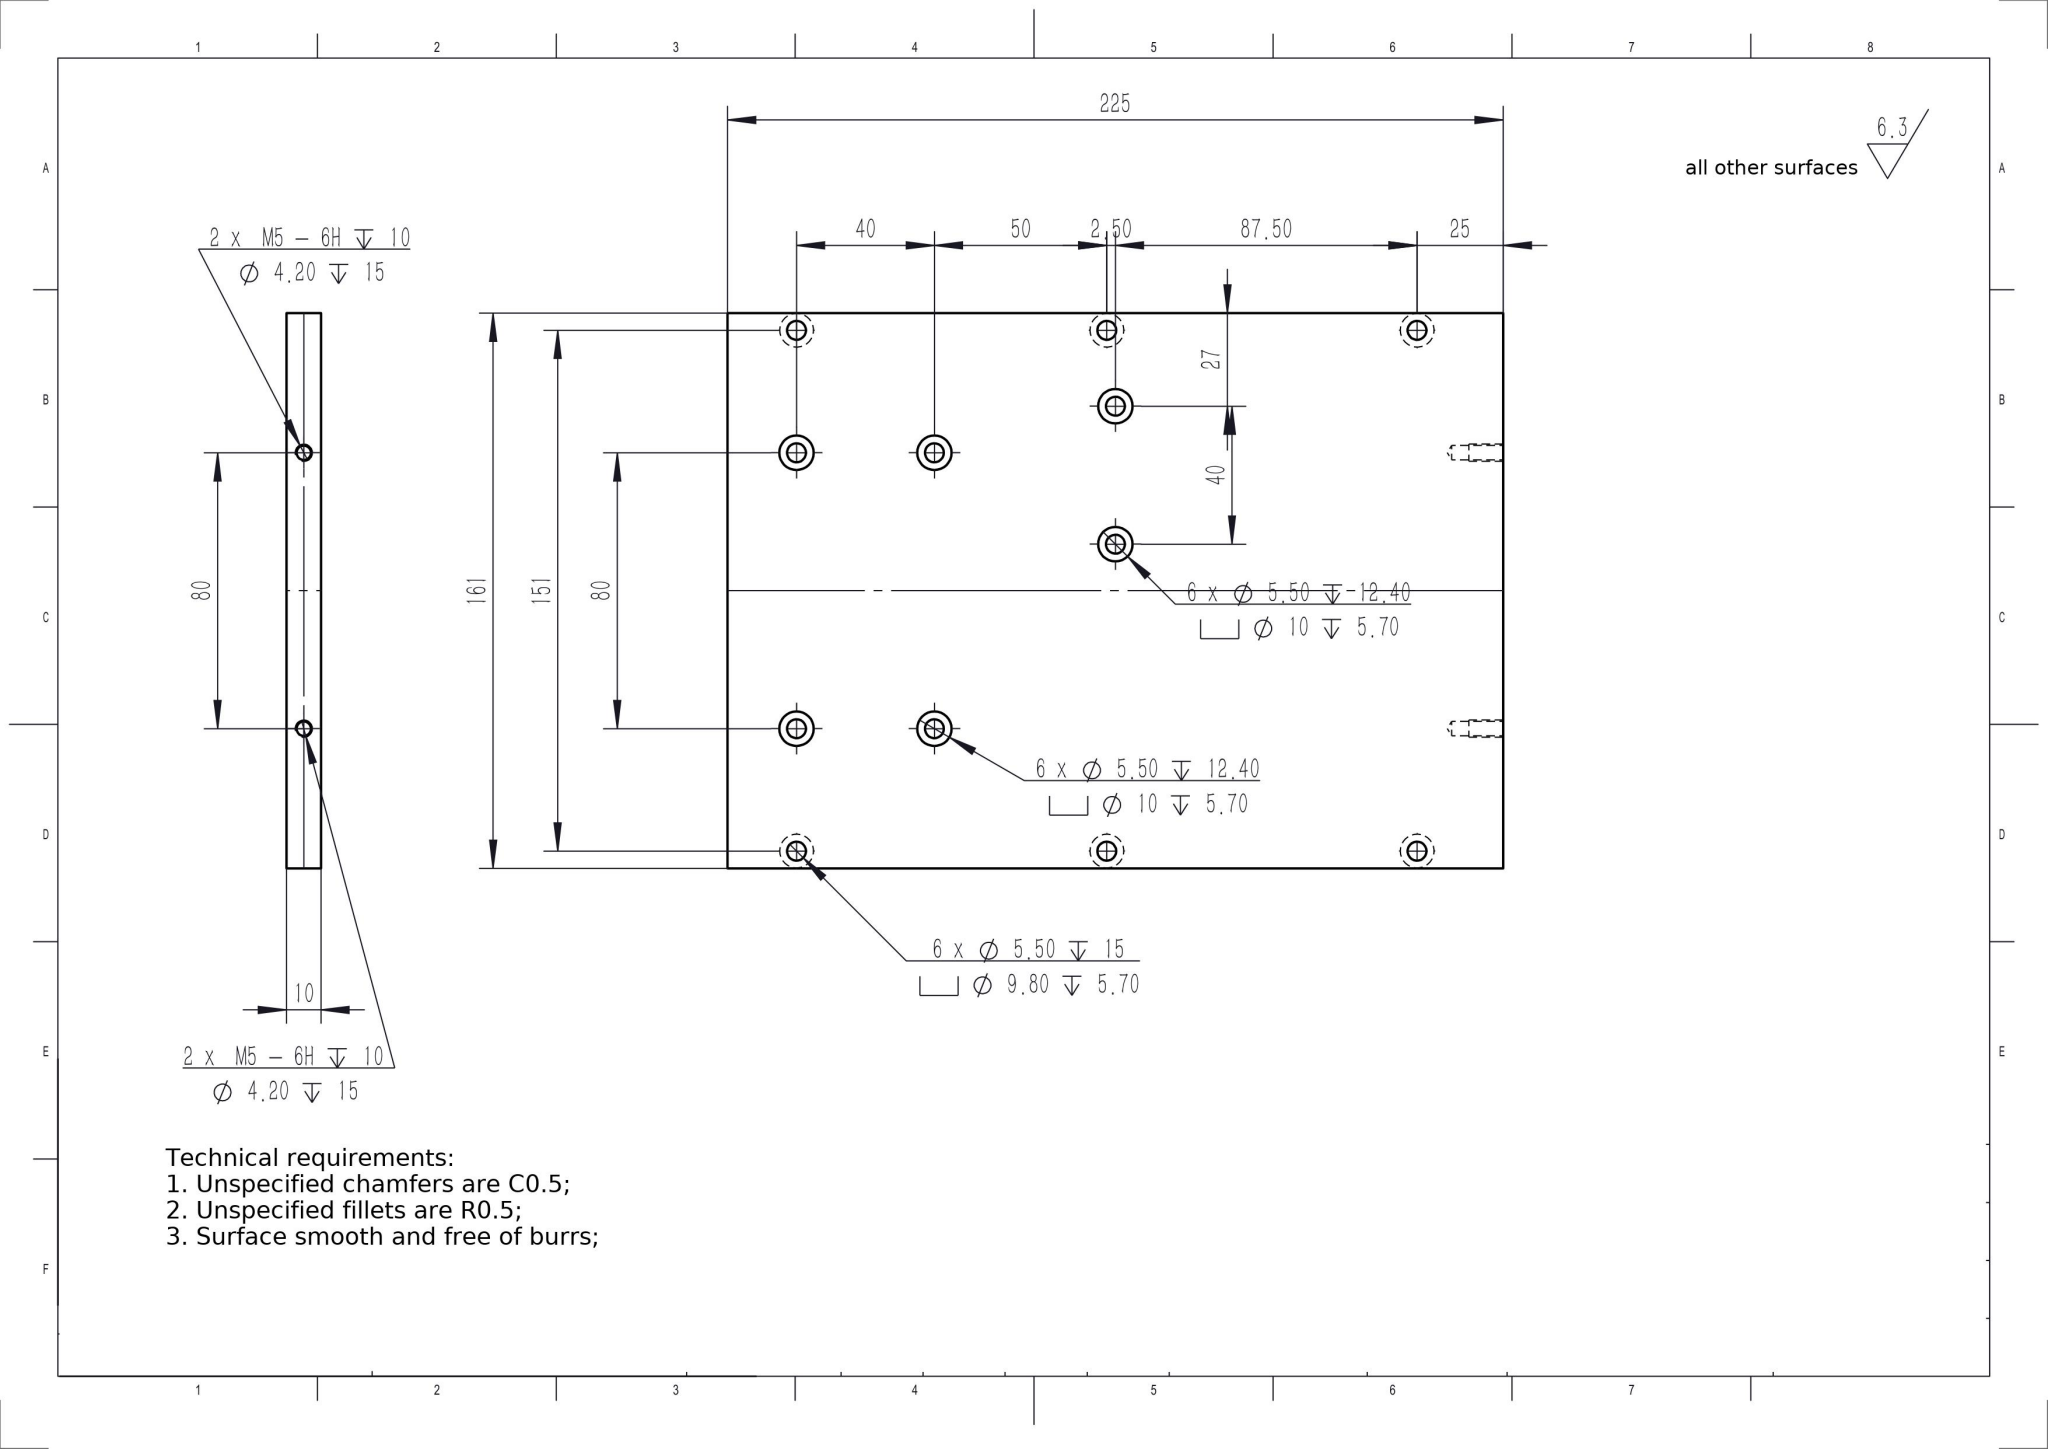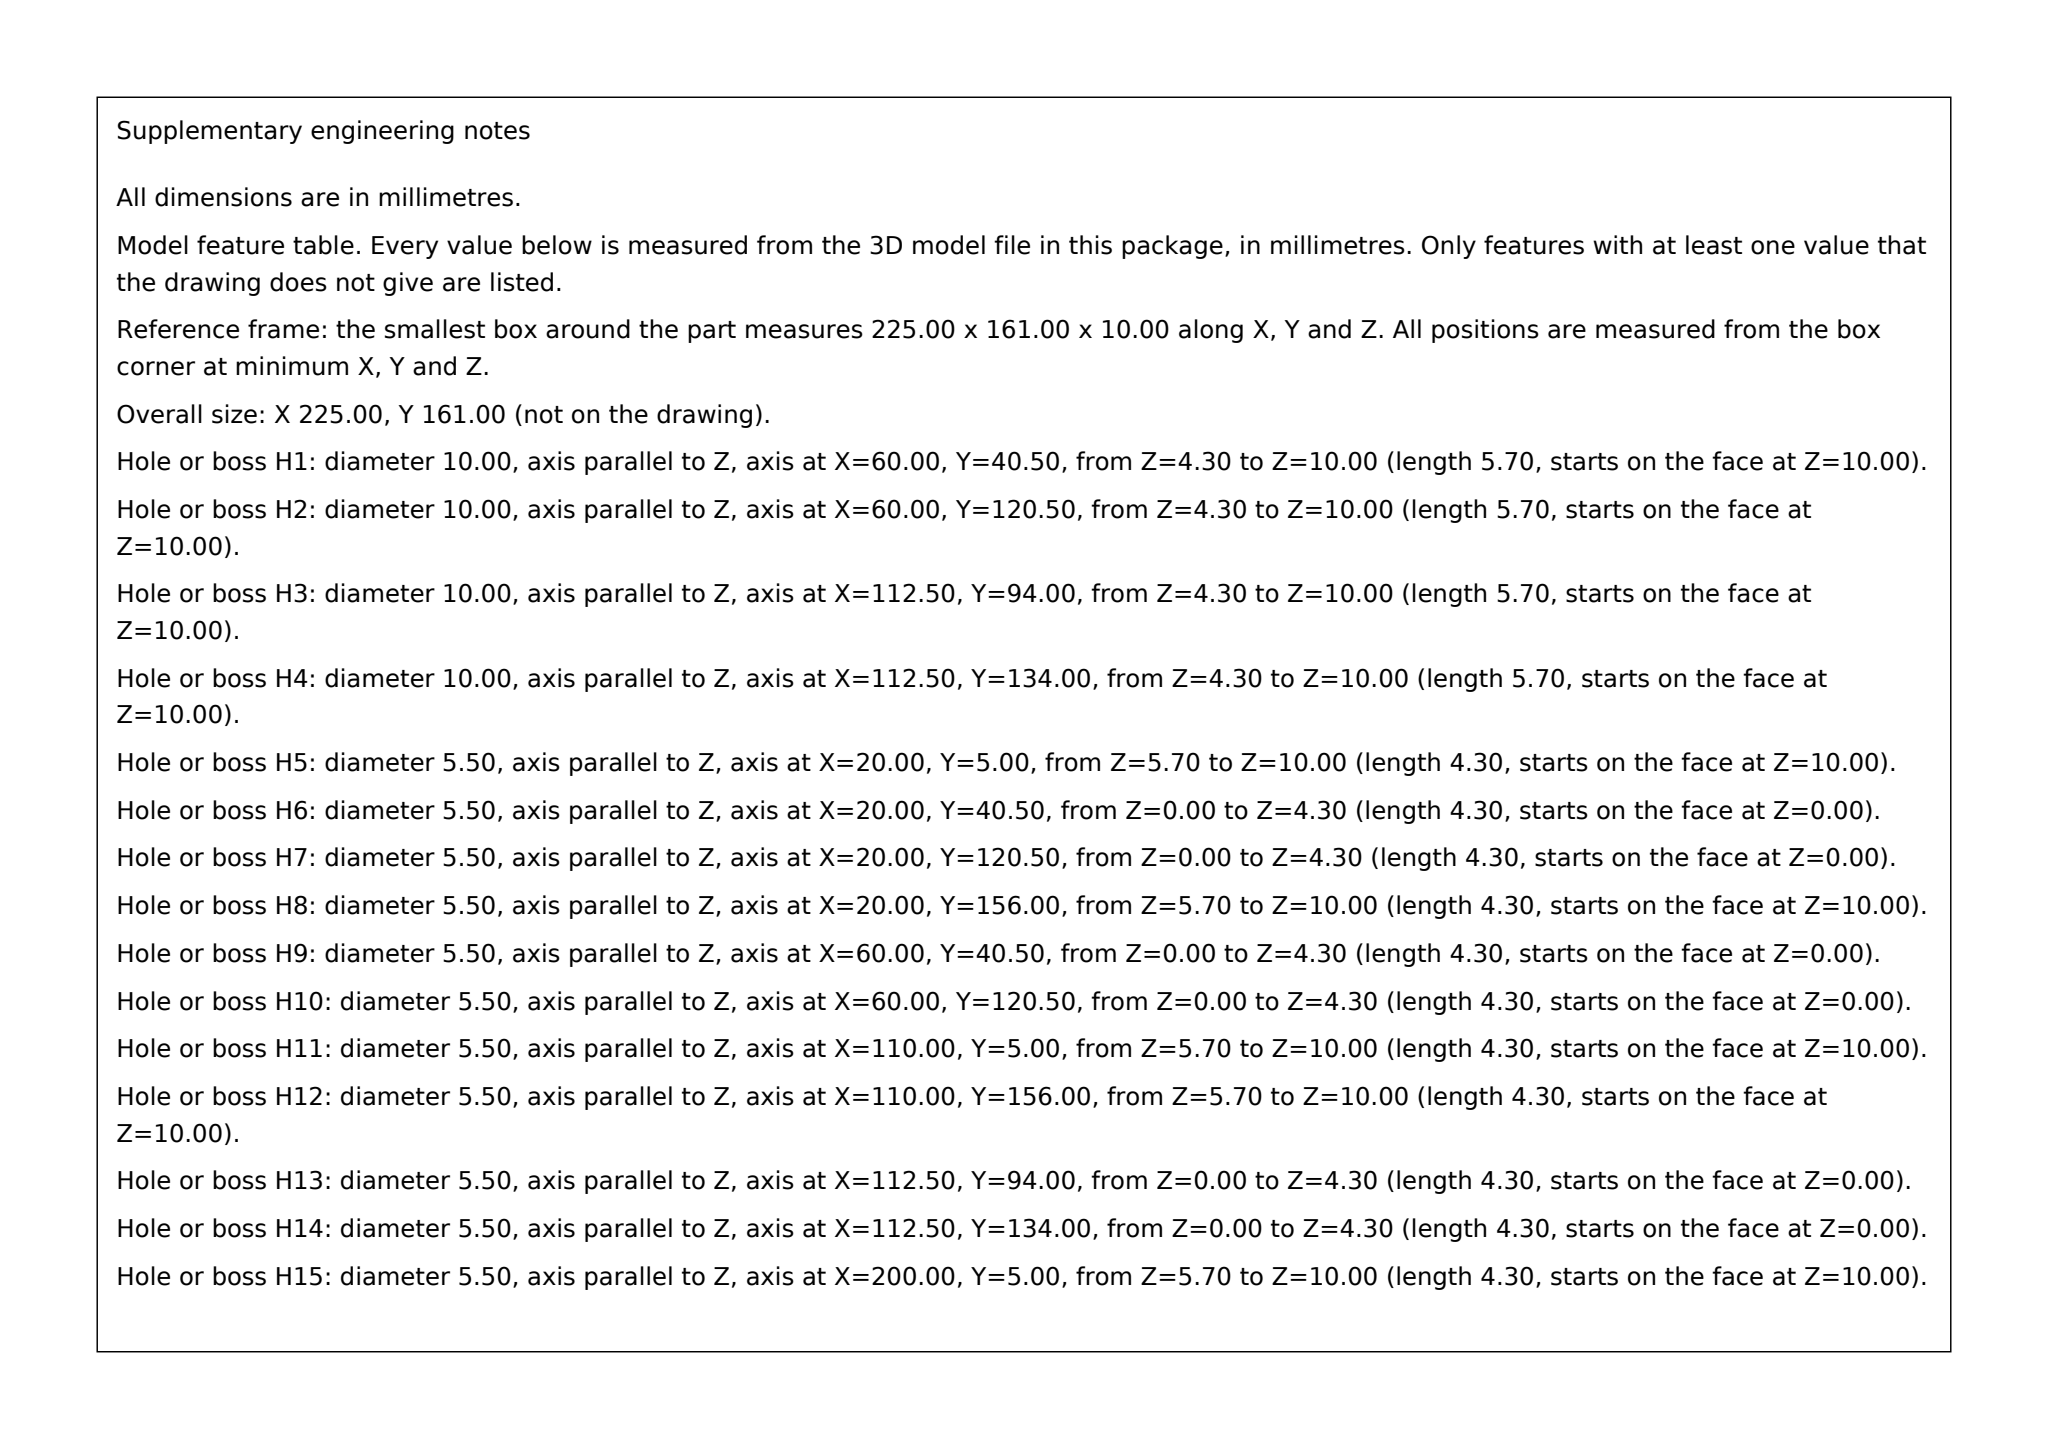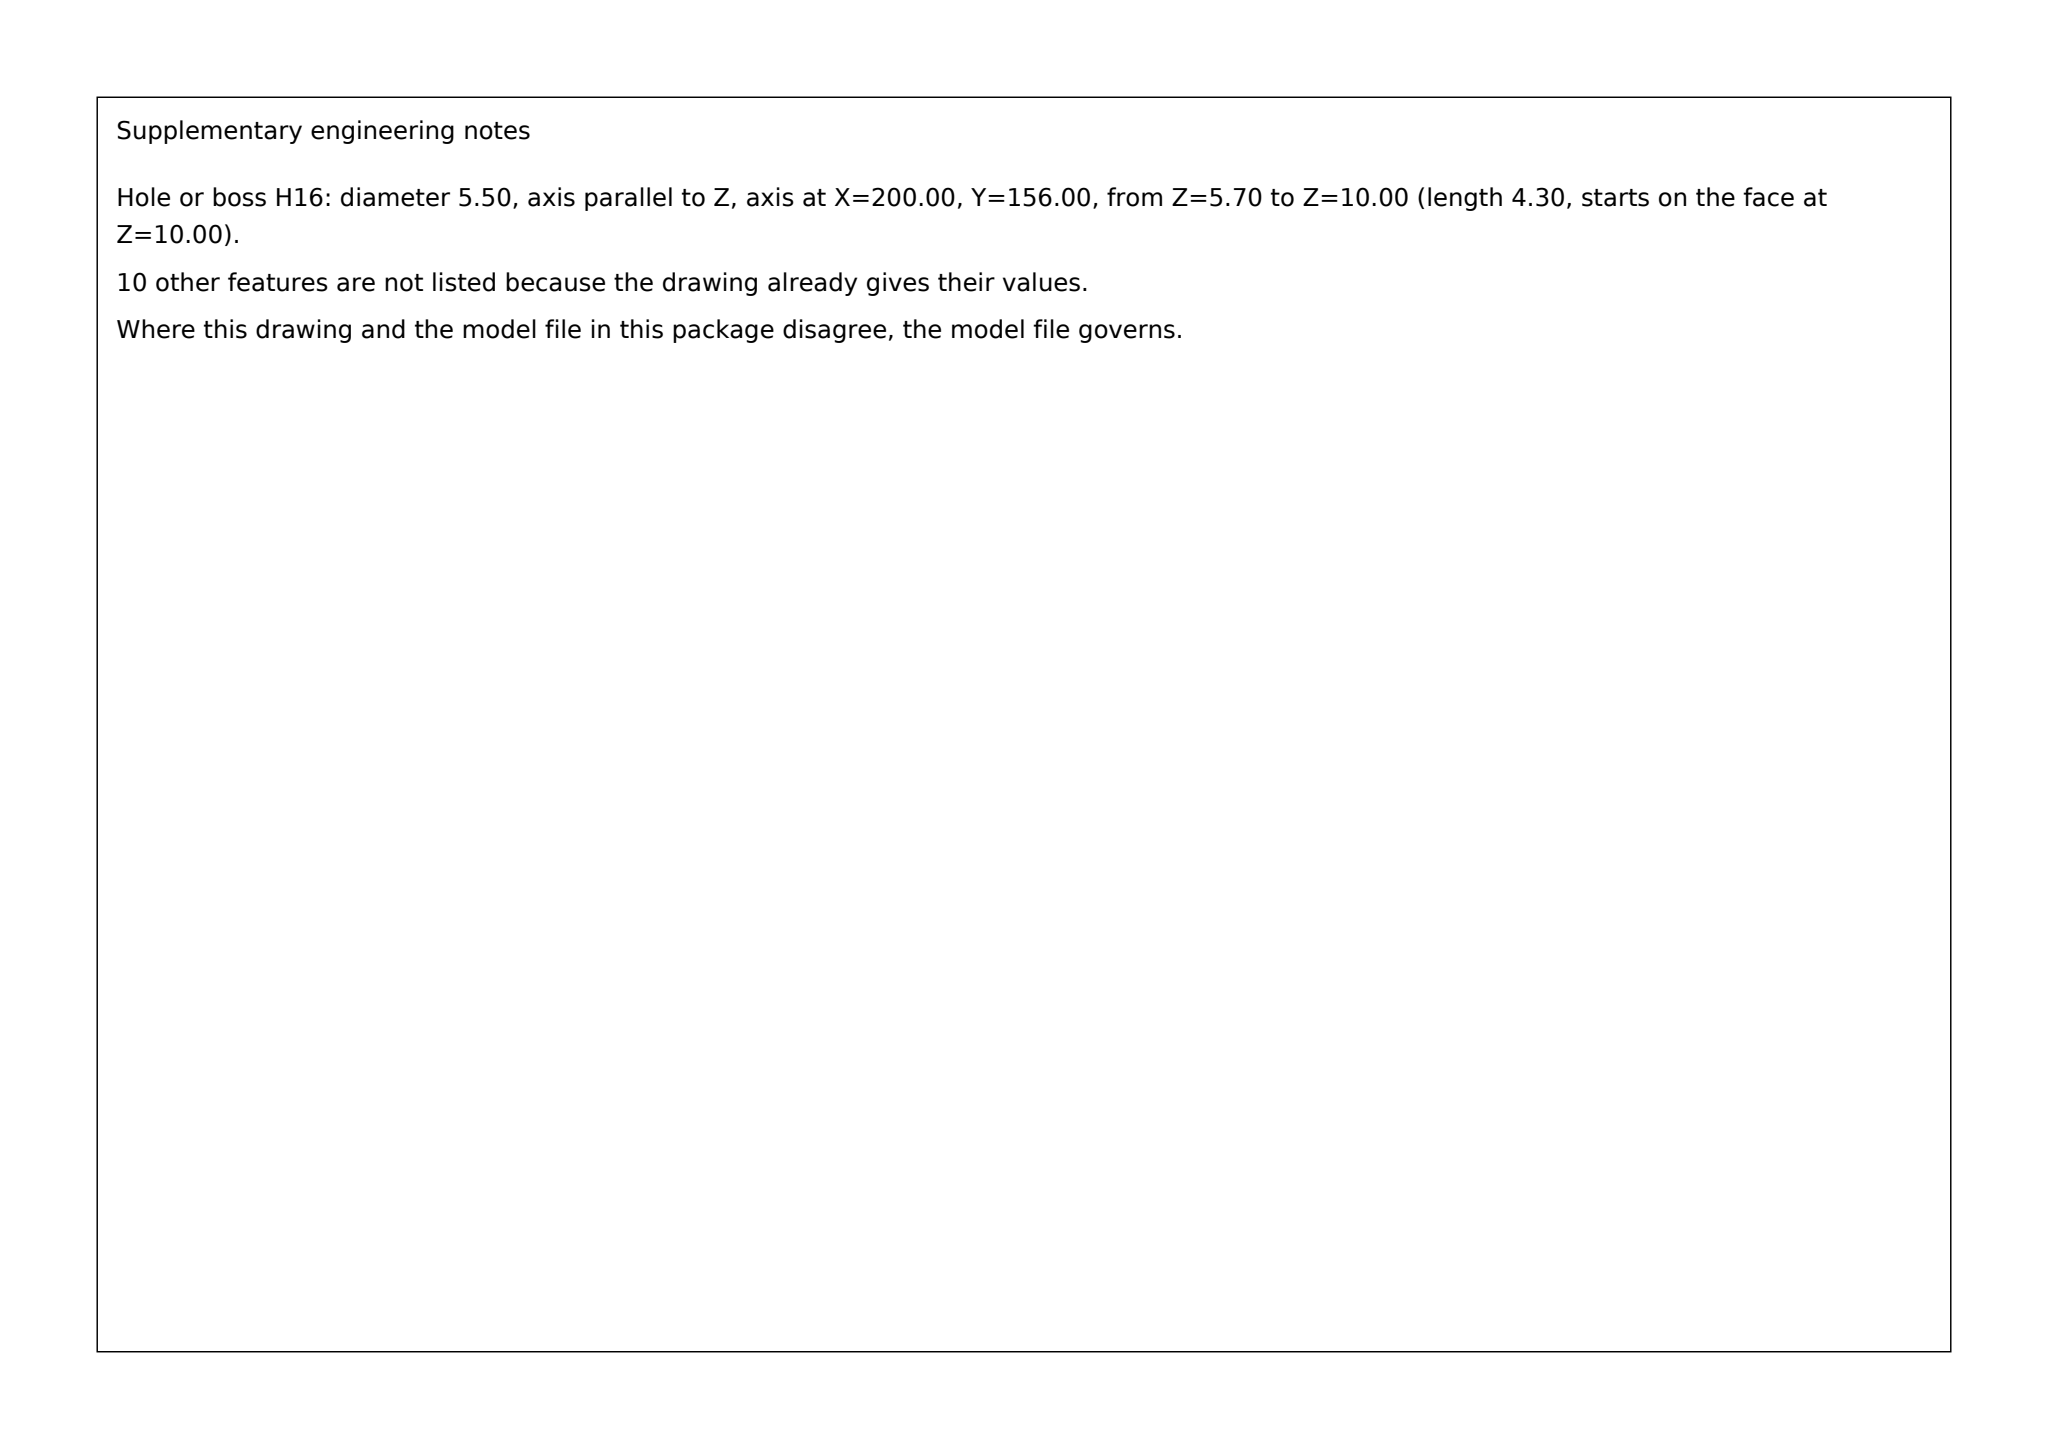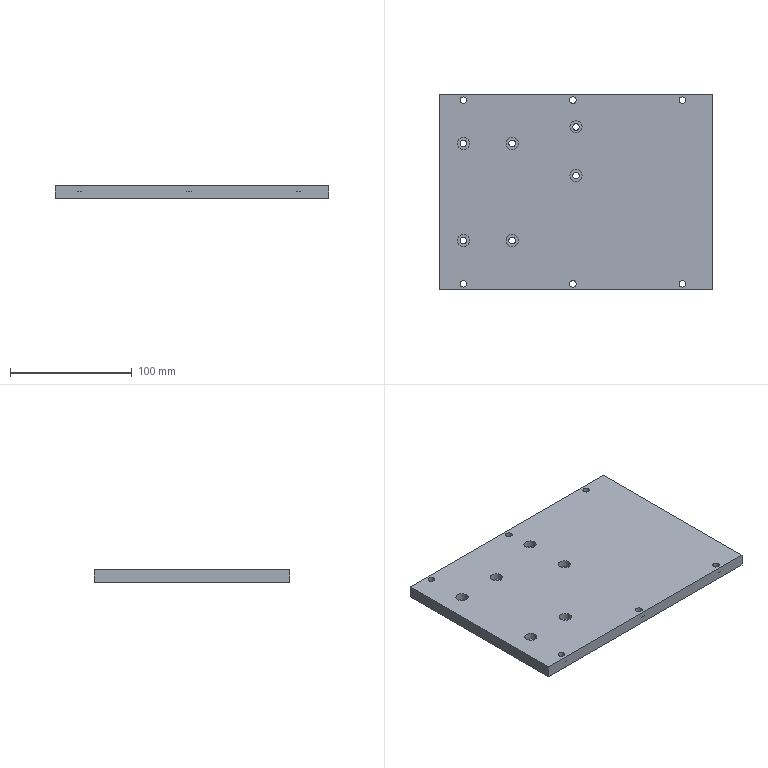Part | SolidWorks | mm | 1 solid | 74 faces | box 225 x 161 x 10 mm | volume 355331 mm3 | cylinder 52 | plane 18 | cone 4 | commonest cylinder face diameters 5.5 x24 10 x12 9.8 x12 4.2 x4
build123d program:
from build123d import *

# Parameters (mm, degrees)
SKETCH1_W                                         = 225
SKETCH1_H                                         = 161
BOSS_EXTRUDE1_DEPTH                               = 10
HOLE_SIZE_ACCORDING_TO_TYPE_OF_HEX_SO_D           = 5.5
HOLE_SIZE_ACCORDING_TO_TYPE_OF_HEX_SO_DEPTH       = 15
HOLE_SIZE_ACCORDING_TO_TYPE_OF_HEX_SO_CBORE_D     = 9.8
HOLE_SIZE_ACCORDING_TO_TYPE_OF_HEX_SO_CBORE_DEPTH = 5.7
HOLE_SIZE_ACCORDING_TO_TYPE_OF_HEX_SO_TIP         = 1.652
M5_TAPPED_HOLE1_D                                 = 4.2
M5_TAPPED_HOLE1_DEPTH                             = 15
M5_TAPPED_HOLE1_TIP                               = 1.262
HOLE_SIZE_ACCORDING_TO_TYPE_OF_HE_2_D             = 5.5
HOLE_SIZE_ACCORDING_TO_TYPE_OF_HE_2_DEPTH         = 12.4
HOLE_SIZE_ACCORDING_TO_TYPE_OF_HE_2_CBORE_D       = 10
HOLE_SIZE_ACCORDING_TO_TYPE_OF_HE_2_CBORE_DEPTH   = 5.7
HOLE_SIZE_ACCORDING_TO_TYPE_OF_HE_2_TIP           = 1.652


with BuildPart() as part:
    # Sketch1 → Boss-Extrude1 (new body)
    with BuildSketch(Plane.XY):
        Rectangle(SKETCH1_W, SKETCH1_H)
    extrude(amount=BOSS_EXTRUDE1_DEPTH)

    # Hole Size _ according to_ type of Hex So
    with Locations(Plane(origin=(0, 0, 0), x_dir=(1, 0, 0), z_dir=(0, 0, -1))):
        with Locations((-92.5, -75.5), (-2.5, -75.5), (87.5, -75.5), (87.5, 75.5), (-2.5, 75.5), (-92.5, 75.5)):
            CounterBoreHole(HOLE_SIZE_ACCORDING_TO_TYPE_OF_HEX_SO_D / 2, HOLE_SIZE_ACCORDING_TO_TYPE_OF_HEX_SO_CBORE_D / 2, HOLE_SIZE_ACCORDING_TO_TYPE_OF_HEX_SO_CBORE_DEPTH, depth=HOLE_SIZE_ACCORDING_TO_TYPE_OF_HEX_SO_DEPTH)
            with Locations((0, 0, -(HOLE_SIZE_ACCORDING_TO_TYPE_OF_HEX_SO_DEPTH + HOLE_SIZE_ACCORDING_TO_TYPE_OF_HEX_SO_TIP / 2))):  # 118° drill point
                Cone(0, HOLE_SIZE_ACCORDING_TO_TYPE_OF_HEX_SO_D / 2, HOLE_SIZE_ACCORDING_TO_TYPE_OF_HEX_SO_TIP, mode=Mode.SUBTRACT)

    # M5 Tapped Hole1
    with Locations(Plane(origin=(112.5, 0, 0), x_dir=(0, 0, -1), z_dir=(1, 0, 0))):
        with Locations((-5, -40), (-5, 40)):
            Hole(M5_TAPPED_HOLE1_D / 2, depth=M5_TAPPED_HOLE1_DEPTH)
            with Locations((0, 0, -(M5_TAPPED_HOLE1_DEPTH + M5_TAPPED_HOLE1_TIP / 2))):  # 118° drill point
                Cone(0, M5_TAPPED_HOLE1_D / 2, M5_TAPPED_HOLE1_TIP, mode=Mode.SUBTRACT)

    # Hole Size _ according to_ type of He 2
    with Locations(Plane.XY.offset(10)):
        with Locations((0, 53.5), (0, 13.5), (-92.5, 40), (-52.5, 40), (-52.5, -40), (-92.5, -40)):
            CounterBoreHole(HOLE_SIZE_ACCORDING_TO_TYPE_OF_HE_2_D / 2, HOLE_SIZE_ACCORDING_TO_TYPE_OF_HE_2_CBORE_D / 2, HOLE_SIZE_ACCORDING_TO_TYPE_OF_HE_2_CBORE_DEPTH, depth=HOLE_SIZE_ACCORDING_TO_TYPE_OF_HE_2_DEPTH)
            with Locations((0, 0, -(HOLE_SIZE_ACCORDING_TO_TYPE_OF_HE_2_DEPTH + HOLE_SIZE_ACCORDING_TO_TYPE_OF_HE_2_TIP / 2))):  # 118° drill point
                Cone(0, HOLE_SIZE_ACCORDING_TO_TYPE_OF_HE_2_D / 2, HOLE_SIZE_ACCORDING_TO_TYPE_OF_HE_2_TIP, mode=Mode.SUBTRACT)


solid = part.part